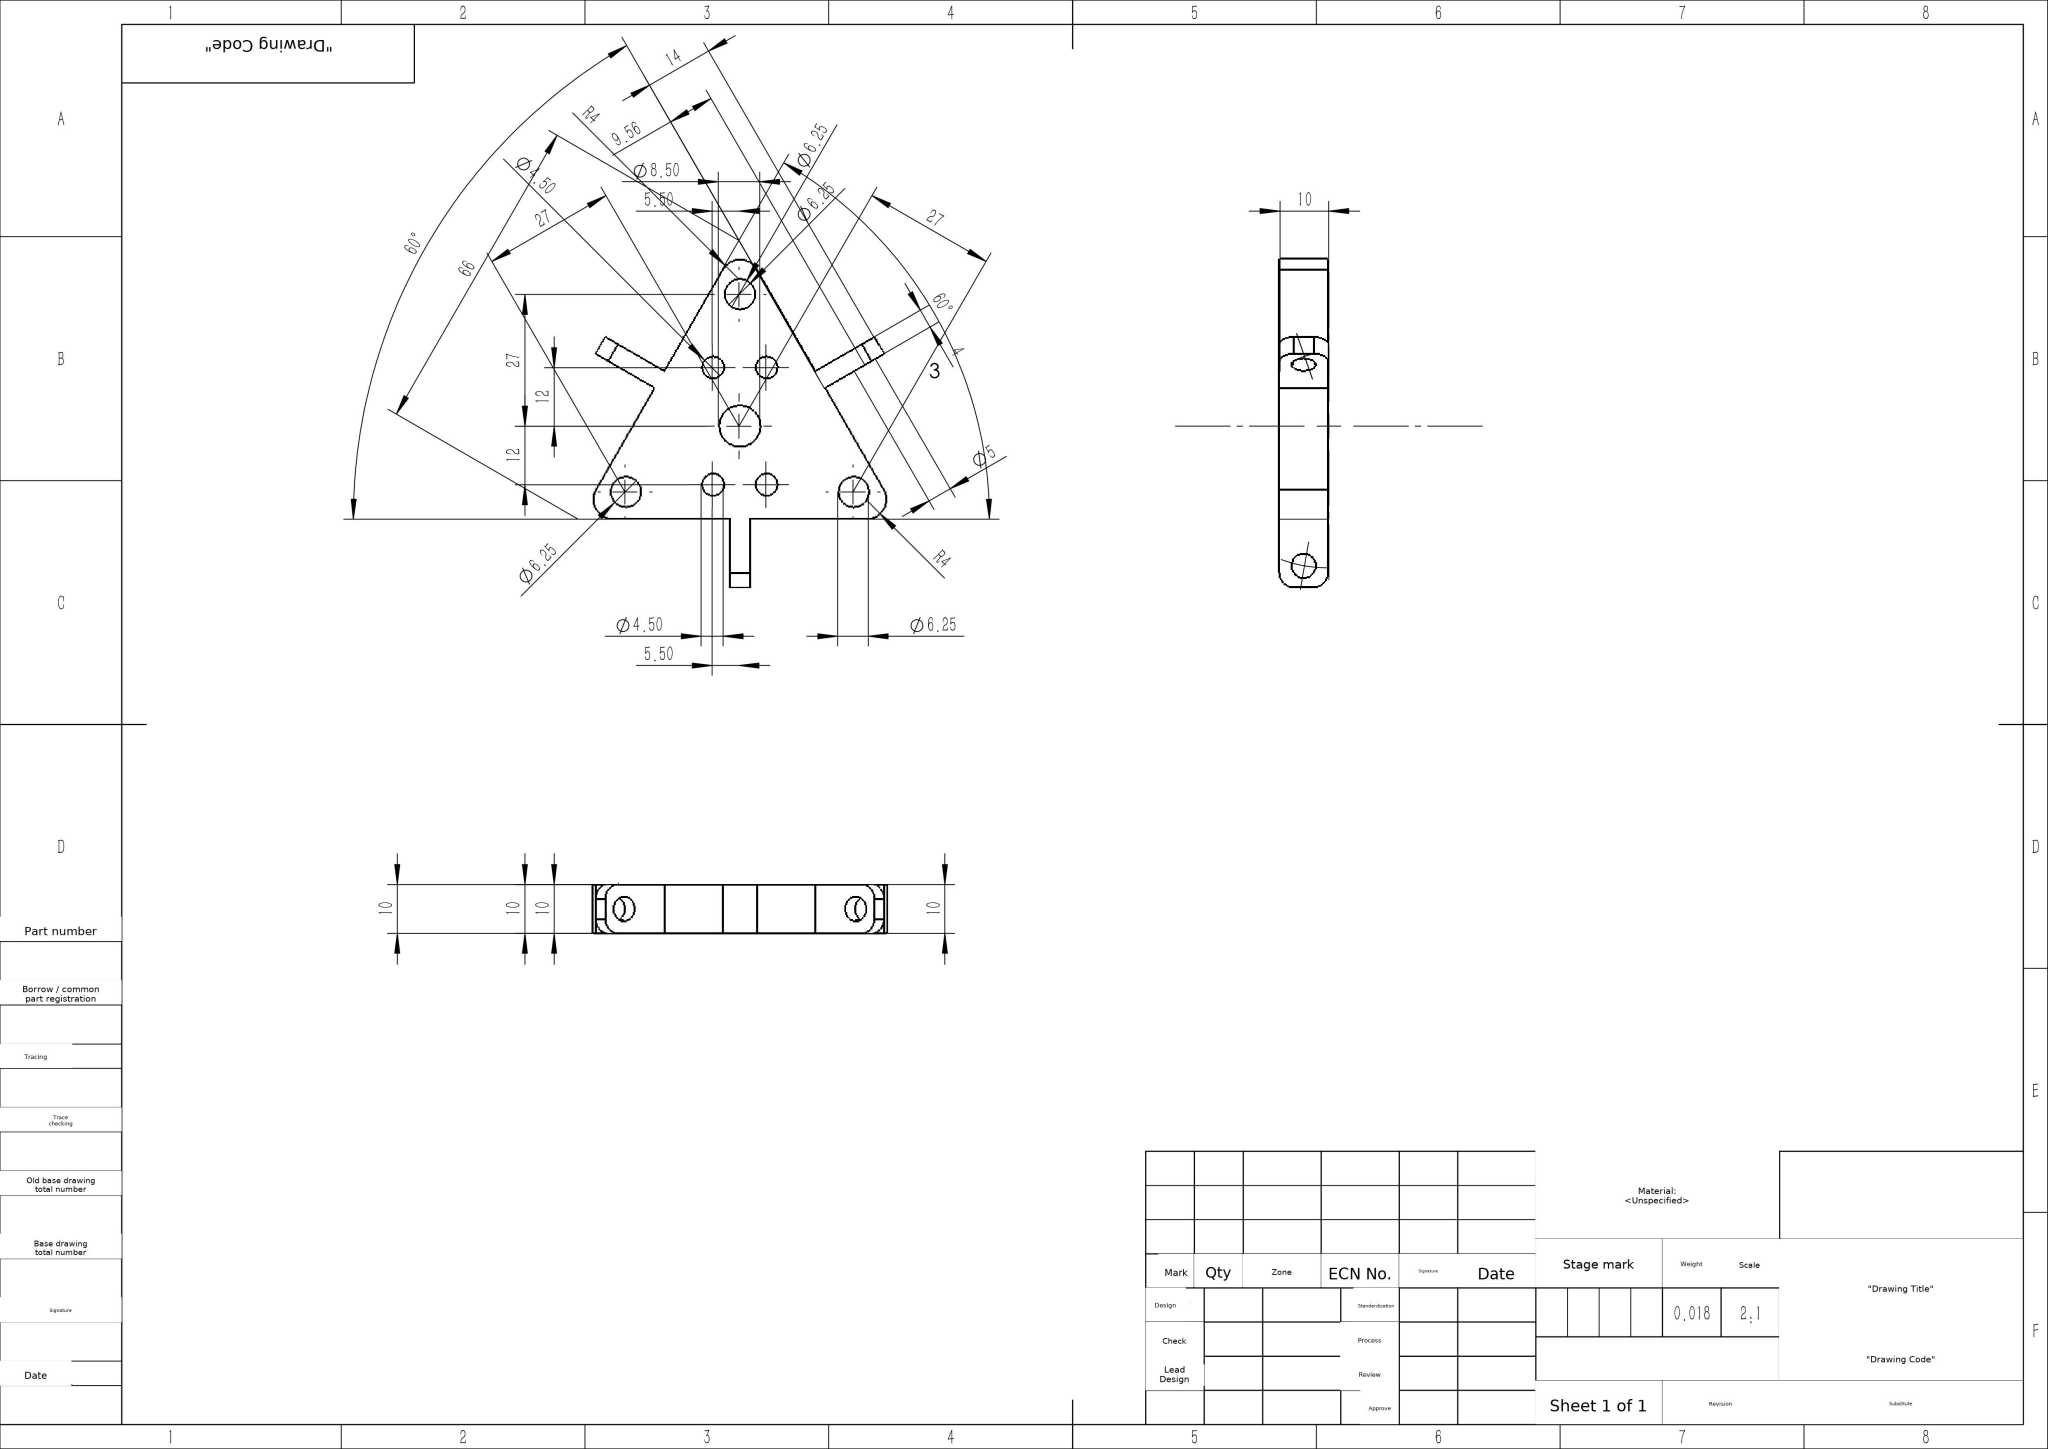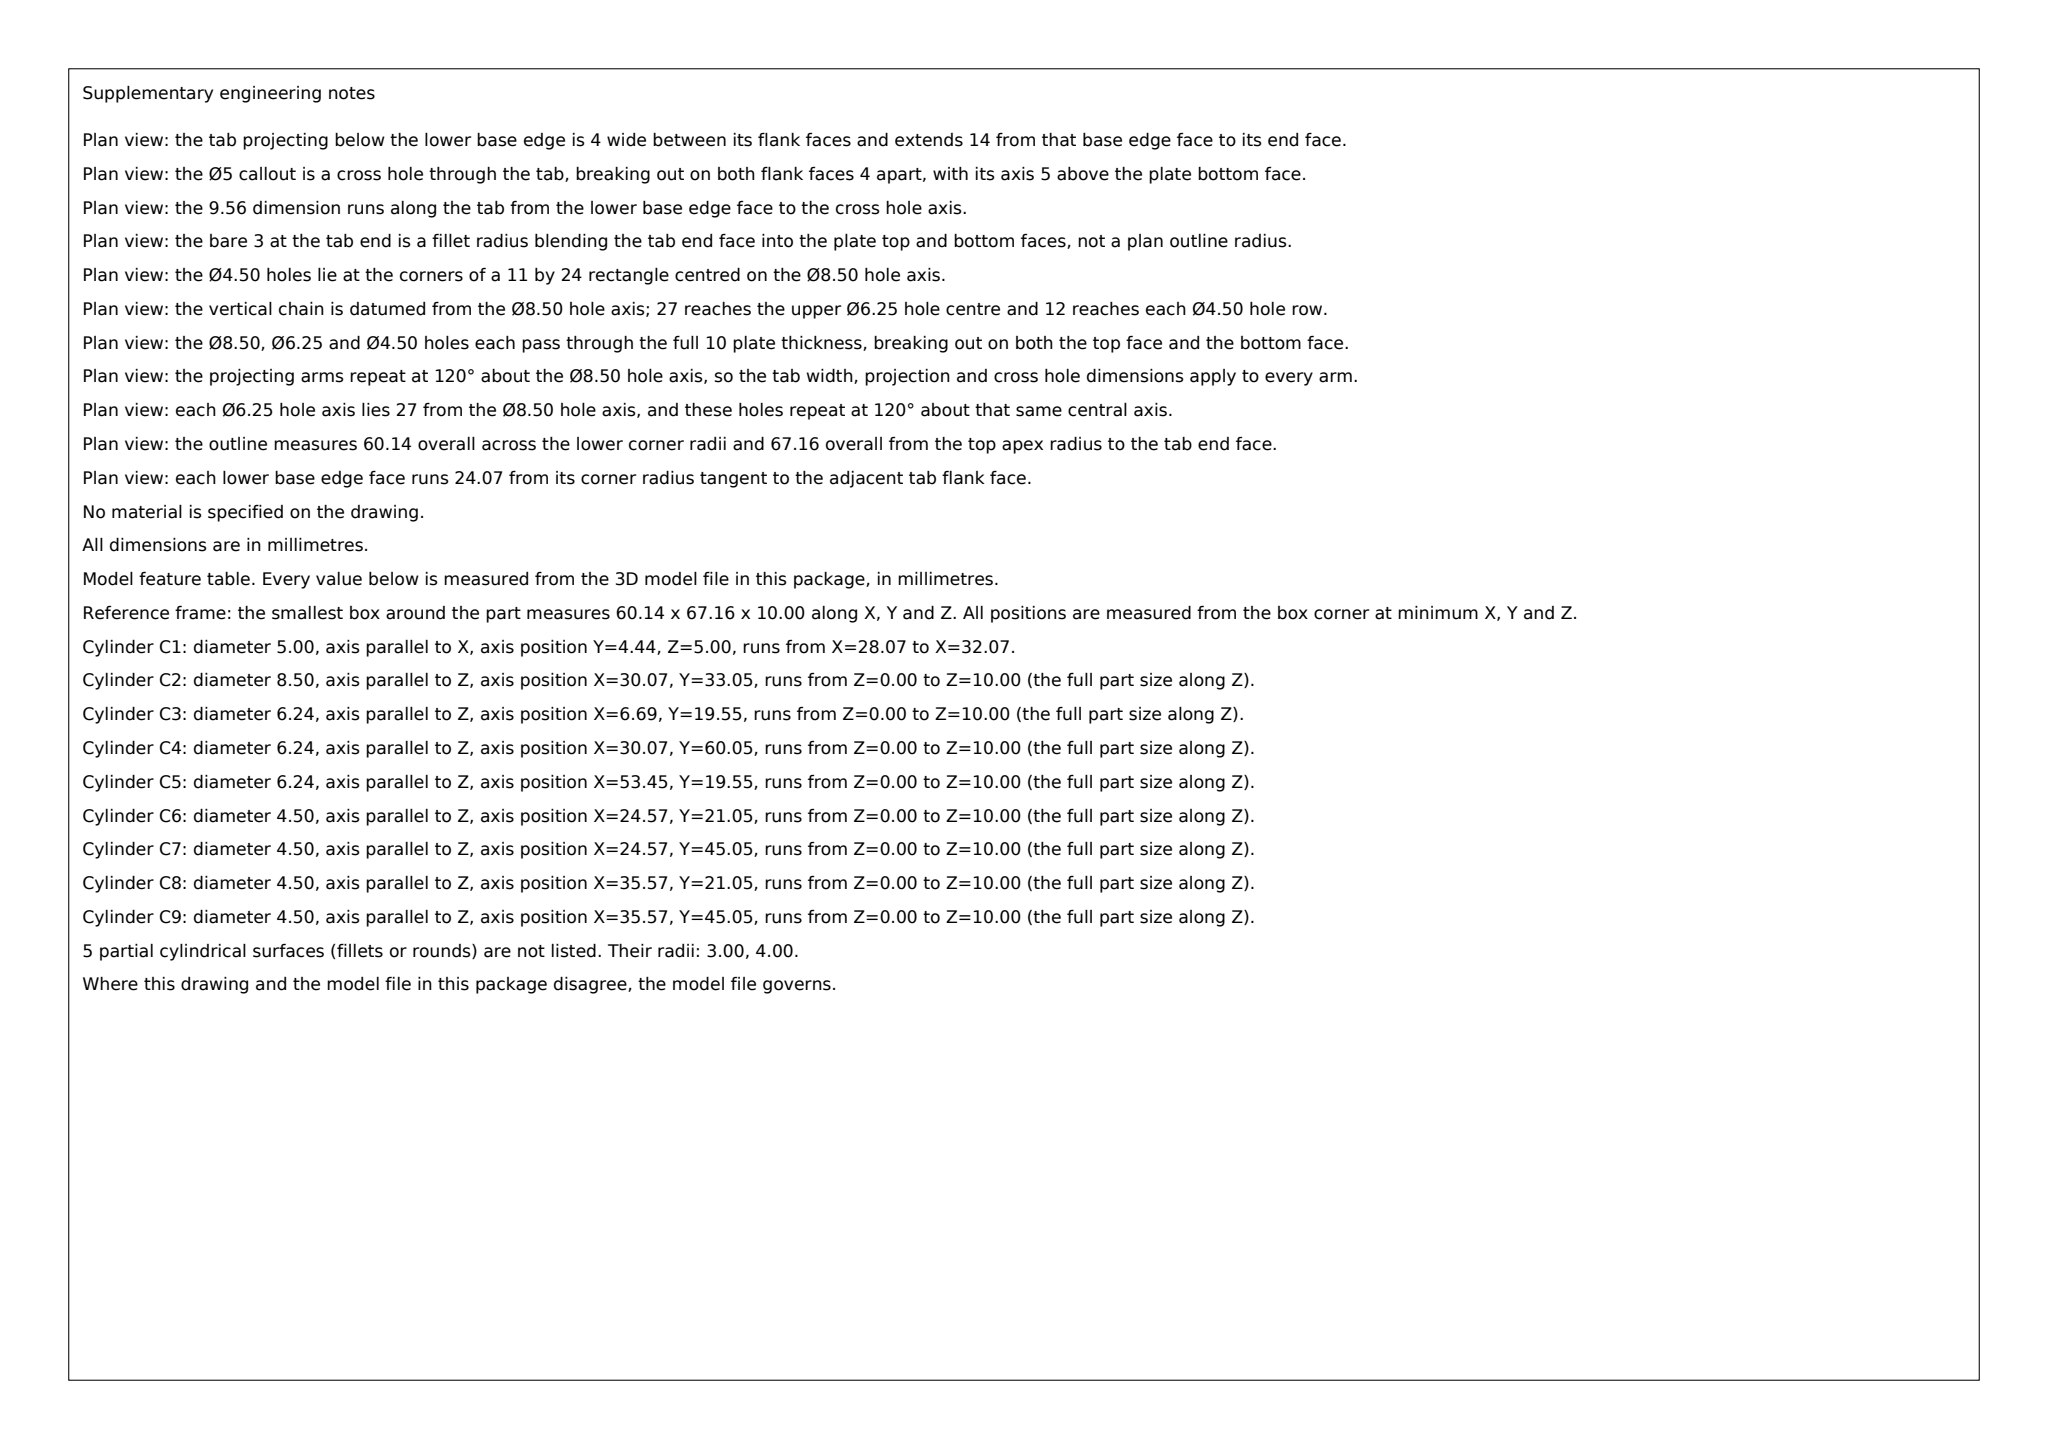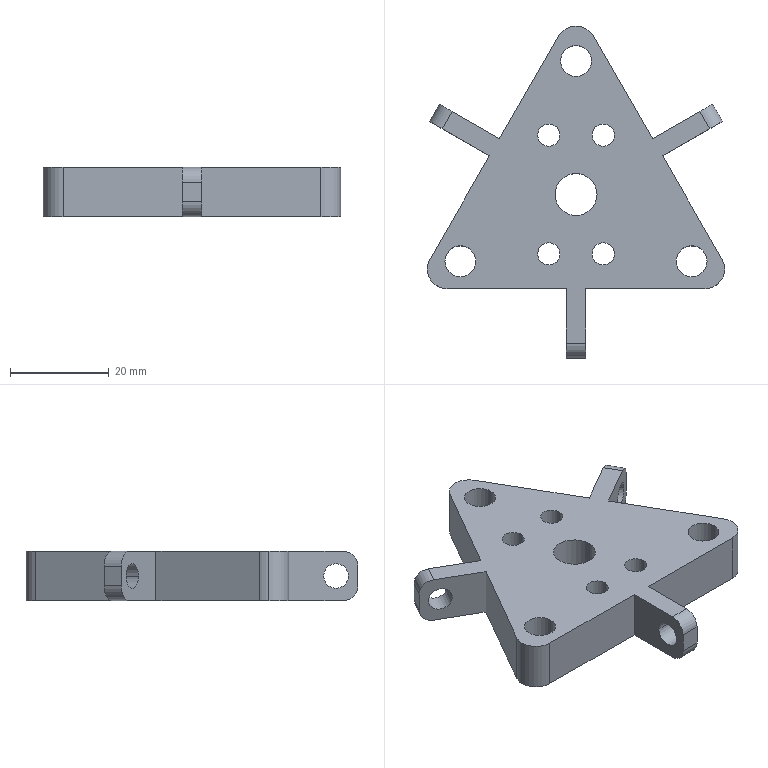Part | SolidWorks | mm | 1 solid | 49 faces | box 60.14 x 67.16 x 10 mm | volume 17807 mm3 | cylinder 32 | plane 17 | commonest cylinder face diameters 4.5 x8 5 x6 6.25 x6 6 x6 8 x4 8.5 x2
Drawing notes:
Overall plate outline 60.14 wide x 67.16 high x 10 thick (datum: lower-left corner of part). | from the solid: bbox_xyz [60.144, 67.158, 10.0]
Central Ø8.50 THRU hole located X 30.07 from left edge, Y 33.05 from bottom edge. | from the solid: cylinder [8.5,z,(30.07,33.05),10.0]
3X Ø6.25 THRU holes at (X 6.69, Y 19.55), (X 30.07, Y 60.05) and (X 53.45, Y 19.55) from lower-left corner. | from the solid: cylinders [6.25,z,(6.69,19.55)], [6.25,z,(30.07,60.05)], [6.25,z,(53.45,19.55)]
4X Ø4.50 THRU holes at X 24.57 and X 35.57, Y 21.05 and Y 45.05 from lower-left corner. | from the solid: cylinders [4.5,z,(24.57,21.05)], [4.5,z,(24.57,45.05)], [4.5,z,(35.57,21.05)], [4.5,z,(35.57,45.05)]
3X R4 arm-end arcs are NOT concentric with the Ø6.25 holes; arc centres at (X 4.00, Y 18.00), (X 30.07, Y 63.16) and (X 56.14, Y 18.00). | from the solid: cylinders [8.0,z,(4.0,18.0)], [8.0,z,(30.07,63.16)], [8.0,z,(56.14,18.0)]
Bottom centre notch 4 wide between X 28.07 and X 32.07 (centred on X 30.07), depth 14 from bottom edge Y 0. | from the solid: axis_planes x=28.07, x=32.07, y=0.0, y=14.0
2X Ø6 bore, axis parallel to X, at Y 3.00, Z 3.00 and Z 7.00, bore length 4. | from the solid: cylinders [6.0,x,(y3.0,z3.0),4.0] and [6.0,x,(y3.0,z7.0),4.0]
4X Ø6 bore, axis parallel to Y, at X 0.04 and X 52.09, Z 3.00 and Z 7.00, bore length 4.96. | from the solid: cylinders [6.0,y,(0.04,z3.0)], [6.0,y,(0.04,z7.0)], [6.0,y,(52.09,z3.0)], [6.0,y,(52.09,z7.0)], length 4.96
Ø5 side feature, axis parallel to X, at Y 4.44, Z 5.00, length 4. | from the solid: cylinder [5.0,x,(y4.44,z5.0),4.0]
2X Ø5 side feature, axis parallel to Y, at X -0.71 and X 48.85, Z 5.00, length 5.96. | from the solid: cylinders [5.0,y,(-0.71,z5.0),5.96] and [5.0,y,(48.85,z5.0),5.96]
All hole and arc locations above are dimensioned from the lower-left corner of the part (X from left edge, Y from bottom edge, Z from bottom face at Z 0, top face Z 10). | from the solid: origin_note: positions are from min corner of bbox; axis_planes z=0.0, z=10.0
ALL DIMENSIONS IN MILLIMETRES. | from the solid: STEP model units: mm
NO FILLETS OR ROUNDS ON INTERNAL CORNERS IN THE MODEL; EDGES SHARP UNLESS OTHERWISE SPECIFIED. | from the solid: fillet_radii: [] (empty)